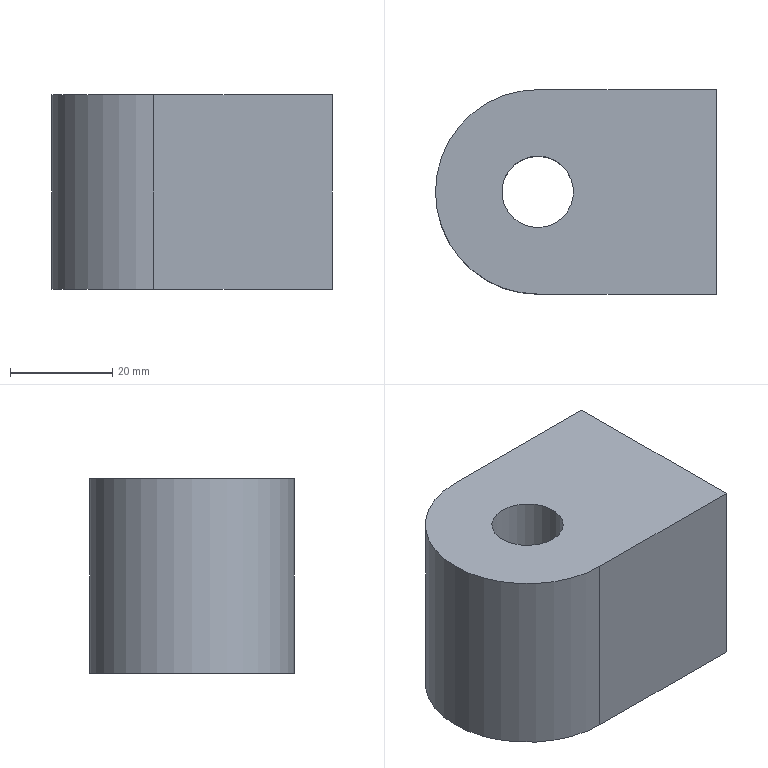Component | NX | Z_AXIS_LEADSCREW_NUT | 1 solid | 15 faces | box 55 x 40 x 38 mm | volume 69853 mm3 | cylinder 6 | plane 5 | cone 4 | commonest cylinder face diameters 5 x4 40 x1 14 x1
STEP:
#1=CARTESIAN_POINT('',(0.,0.,0.));
#2=DIRECTION('',(0.,0.,1.));
#3=DIRECTION('',(1.,0.,0.));
#4=AXIS2_PLACEMENT_3D('',#1,#2,#3);
#5=CARTESIAN_POINT('',(660.689,-130.302,-1073.));
#6=VERTEX_POINT('',#5);
#7=CARTESIAN_POINT('',(625.689,-130.302,-1073.));
#8=VERTEX_POINT('',#7);
#9=CARTESIAN_POINT('',(660.689,-130.302,-1073.));
#10=DIRECTION('',(-1.,0.,0.));
#11=VECTOR('',#10,1.);
#12=LINE('',#9,#11);
#13=CARTESIAN_POINT('',(660.689,-130.302,-1035.));
#14=DIRECTION('',(0.,-1.,0.));
#15=DIRECTION('',(0.,0.,-1.));
#16=AXIS2_PLACEMENT_3D('',#13,#14,#15);
#17=PLANE('',#16);
#18=CARTESIAN_POINT('',(38.,0.));
#19=DIRECTION('',(0.,-1.));
#20=VECTOR('',#19,1.);
#21=LINE('',#18,#20);
#22=(GEOMETRIC_REPRESENTATION_CONTEXT(2)PARAMETRIC_REPRESENTATION_CONTEXT()REPRESENTATION_CONTEXT('',''));
#23=DEFINITIONAL_REPRESENTATION('',(#21),#22);
#24=PCURVE('',#17,#23);
#25=CARTESIAN_POINT('',(625.689,-150.302,-1073.));
#26=DIRECTION('',(0.,0.,1.));
#27=DIRECTION('',(0.,-1.,0.));
#28=AXIS2_PLACEMENT_3D('',#25,#26,#27);
#29=PLANE('',#28);
#30=CARTESIAN_POINT('',(-20.,35.));
#31=DIRECTION('',(0.,-1.));
#32=VECTOR('',#31,1.);
#33=LINE('',#30,#32);
#34=(GEOMETRIC_REPRESENTATION_CONTEXT(2)PARAMETRIC_REPRESENTATION_CONTEXT()REPRESENTATION_CONTEXT('',''));
#35=DEFINITIONAL_REPRESENTATION('',(#33),#34);
#36=PCURVE('',#29,#35);
#37=SURFACE_CURVE('',#12,(#24,#36),.PCURVE_S1.);
#38=EDGE_CURVE('',#6,#8,#37,.T.);
#39=ORIENTED_EDGE('',*,*,#38,.T.);
#40=CARTESIAN_POINT('',(625.689,-130.302,-1035.));
#41=VERTEX_POINT('',#40);
#42=CARTESIAN_POINT('',(625.689,-130.302,-1035.));
#43=DIRECTION('',(0.,0.,-1.));
#44=VECTOR('',#43,1.);
#45=LINE('',#42,#44);
#46=CARTESIAN_POINT('',(0.,-35.));
#47=DIRECTION('',(1.,0.));
#48=VECTOR('',#47,1.);
#49=LINE('',#46,#48);
#50=(GEOMETRIC_REPRESENTATION_CONTEXT(2)PARAMETRIC_REPRESENTATION_CONTEXT()REPRESENTATION_CONTEXT('',''));
#51=DEFINITIONAL_REPRESENTATION('',(#49),#50);
#52=PCURVE('',#17,#51);
#53=CARTESIAN_POINT('',(625.689,-150.302,-1035.));
#54=DIRECTION('',(0.,0.,-1.));
#55=DIRECTION('',(0.,1.,0.));
#56=AXIS2_PLACEMENT_3D('',#53,#54,#55);
#57=CYLINDRICAL_SURFACE('',#56,20.);
#58=CARTESIAN_POINT('',(6.283,0.));
#59=DIRECTION('',(0.,1.));
#60=VECTOR('',#59,1.);
#61=LINE('',#58,#60);
#62=(GEOMETRIC_REPRESENTATION_CONTEXT(2)PARAMETRIC_REPRESENTATION_CONTEXT()REPRESENTATION_CONTEXT('',''));
#63=DEFINITIONAL_REPRESENTATION('',(#61),#62);
#64=PCURVE('',#57,#63);
#65=SURFACE_CURVE('',#45,(#52,#64),.PCURVE_S1.);
#66=EDGE_CURVE('',#41,#8,#65,.T.);
#67=ORIENTED_EDGE('',*,*,#66,.F.);
#68=CARTESIAN_POINT('',(660.689,-130.302,-1035.));
#69=VERTEX_POINT('',#68);
#70=CARTESIAN_POINT('',(660.689,-130.302,-1035.));
#71=DIRECTION('',(-1.,0.,0.));
#72=VECTOR('',#71,1.);
#73=LINE('',#70,#72);
#74=CARTESIAN_POINT('',(0.,0.));
#75=DIRECTION('',(0.,-1.));
#76=VECTOR('',#75,1.);
#77=LINE('',#74,#76);
#78=(GEOMETRIC_REPRESENTATION_CONTEXT(2)PARAMETRIC_REPRESENTATION_CONTEXT()REPRESENTATION_CONTEXT('',''));
#79=DEFINITIONAL_REPRESENTATION('',(#77),#78);
#80=PCURVE('',#17,#79);
#81=CARTESIAN_POINT('',(625.689,-150.302,-1035.));
#82=DIRECTION('',(0.,0.,1.));
#83=DIRECTION('',(0.,-1.,0.));
#84=AXIS2_PLACEMENT_3D('',#81,#82,#83);
#85=PLANE('',#84);
#86=CARTESIAN_POINT('',(-20.,35.));
#87=DIRECTION('',(0.,-1.));
#88=VECTOR('',#87,1.);
#89=LINE('',#86,#88);
#90=(GEOMETRIC_REPRESENTATION_CONTEXT(2)PARAMETRIC_REPRESENTATION_CONTEXT()REPRESENTATION_CONTEXT('',''));
#91=DEFINITIONAL_REPRESENTATION('',(#89),#90);
#92=PCURVE('',#85,#91);
#93=SURFACE_CURVE('',#73,(#80,#92),.PCURVE_S1.);
#94=EDGE_CURVE('',#69,#41,#93,.T.);
#95=ORIENTED_EDGE('',*,*,#94,.F.);
#96=CARTESIAN_POINT('',(660.689,-130.302,-1035.));
#97=DIRECTION('',(0.,0.,-1.));
#98=VECTOR('',#97,1.);
#99=LINE('',#96,#98);
#100=CARTESIAN_POINT('',(0.,0.));
#101=DIRECTION('',(1.,0.));
#102=VECTOR('',#101,1.);
#103=LINE('',#100,#102);
#104=(GEOMETRIC_REPRESENTATION_CONTEXT(2)PARAMETRIC_REPRESENTATION_CONTEXT()REPRESENTATION_CONTEXT('',''));
#105=DEFINITIONAL_REPRESENTATION('',(#103),#104);
#106=PCURVE('',#17,#105);
#107=CARTESIAN_POINT('',(660.689,-170.302,-1035.));
#108=DIRECTION('',(-1.,0.,0.));
#109=DIRECTION('',(0.,0.,-1.));
#110=AXIS2_PLACEMENT_3D('',#107,#108,#109);
#111=PLANE('',#110);
#112=CARTESIAN_POINT('',(0.,-40.));
#113=DIRECTION('',(1.,0.));
#114=VECTOR('',#113,1.);
#115=LINE('',#112,#114);
#116=(GEOMETRIC_REPRESENTATION_CONTEXT(2)PARAMETRIC_REPRESENTATION_CONTEXT()REPRESENTATION_CONTEXT('',''));
#117=DEFINITIONAL_REPRESENTATION('',(#115),#116);
#118=PCURVE('',#111,#117);
#119=SURFACE_CURVE('',#99,(#106,#118),.PCURVE_S1.);
#120=EDGE_CURVE('',#69,#6,#119,.T.);
#121=ORIENTED_EDGE('',*,*,#120,.T.);
#122=EDGE_LOOP('',(#39,#67,#95,#121));
#123=FACE_BOUND('',#122,.T.);
#124=ADVANCED_FACE('',(#123),#17,.F.);
#125=CARTESIAN_POINT('',(625.689,-170.302,-1073.));
#126=VERTEX_POINT('',#125);
#127=CARTESIAN_POINT('',(625.689,-150.302,-1073.));
#128=DIRECTION('',(0.,0.,1.));
#129=DIRECTION('',(0.,-1.,0.));
#130=AXIS2_PLACEMENT_3D('',#127,#128,#129);
#131=CIRCLE('',#130,20.);
#132=CARTESIAN_POINT('',(9.425,38.));
#133=DIRECTION('',(-1.,0.));
#134=VECTOR('',#133,1.);
#135=LINE('',#132,#134);
#136=(GEOMETRIC_REPRESENTATION_CONTEXT(2)PARAMETRIC_REPRESENTATION_CONTEXT()REPRESENTATION_CONTEXT('',''));
#137=DEFINITIONAL_REPRESENTATION('',(#135),#136);
#138=PCURVE('',#57,#137);
#139=CARTESIAN_POINT('',(0.,0.));
#140=DIRECTION('',(1.,0.));
#141=AXIS2_PLACEMENT_2D('',#139,#140);
#142=CIRCLE('',#141,20.);
#143=(GEOMETRIC_REPRESENTATION_CONTEXT(2)PARAMETRIC_REPRESENTATION_CONTEXT()REPRESENTATION_CONTEXT('',''));
#144=DEFINITIONAL_REPRESENTATION('',(#142),#143);
#145=PCURVE('',#29,#144);
#146=SURFACE_CURVE('',#131,(#138,#145),.PCURVE_S1.);
#147=EDGE_CURVE('',#8,#126,#146,.T.);
#148=ORIENTED_EDGE('',*,*,#147,.T.);
#149=CARTESIAN_POINT('',(625.689,-170.302,-1035.));
#150=VERTEX_POINT('',#149);
#151=CARTESIAN_POINT('',(625.689,-170.302,-1035.));
#152=DIRECTION('',(0.,0.,-1.));
#153=VECTOR('',#152,1.);
#154=LINE('',#151,#153);
#155=CARTESIAN_POINT('',(3.142,0.));
#156=DIRECTION('',(0.,1.));
#157=VECTOR('',#156,1.);
#158=LINE('',#155,#157);
#159=(GEOMETRIC_REPRESENTATION_CONTEXT(2)PARAMETRIC_REPRESENTATION_CONTEXT()REPRESENTATION_CONTEXT('',''));
#160=DEFINITIONAL_REPRESENTATION('',(#158),#159);
#161=PCURVE('',#57,#160);
#162=CARTESIAN_POINT('',(625.689,-170.302,-1035.));
#163=DIRECTION('',(0.,1.,0.));
#164=DIRECTION('',(0.,0.,1.));
#165=AXIS2_PLACEMENT_3D('',#162,#163,#164);
#166=PLANE('',#165);
#167=CARTESIAN_POINT('',(0.,0.));
#168=DIRECTION('',(-1.,0.));
#169=VECTOR('',#168,1.);
#170=LINE('',#167,#169);
#171=(GEOMETRIC_REPRESENTATION_CONTEXT(2)PARAMETRIC_REPRESENTATION_CONTEXT()REPRESENTATION_CONTEXT('',''));
#172=DEFINITIONAL_REPRESENTATION('',(#170),#171);
#173=PCURVE('',#166,#172);
#174=SURFACE_CURVE('',#154,(#161,#173),.PCURVE_S1.);
#175=EDGE_CURVE('',#150,#126,#174,.T.);
#176=ORIENTED_EDGE('',*,*,#175,.F.);
#177=CARTESIAN_POINT('',(625.689,-150.302,-1035.));
#178=DIRECTION('',(0.,0.,1.));
#179=DIRECTION('',(0.,-1.,0.));
#180=AXIS2_PLACEMENT_3D('',#177,#178,#179);
#181=CIRCLE('',#180,20.);
#182=CARTESIAN_POINT('',(9.425,0.));
#183=DIRECTION('',(-1.,0.));
#184=VECTOR('',#183,1.);
#185=LINE('',#182,#184);
#186=(GEOMETRIC_REPRESENTATION_CONTEXT(2)PARAMETRIC_REPRESENTATION_CONTEXT()REPRESENTATION_CONTEXT('',''));
#187=DEFINITIONAL_REPRESENTATION('',(#185),#186);
#188=PCURVE('',#57,#187);
#189=CARTESIAN_POINT('',(0.,0.));
#190=DIRECTION('',(1.,0.));
#191=AXIS2_PLACEMENT_2D('',#189,#190);
#192=CIRCLE('',#191,20.);
#193=(GEOMETRIC_REPRESENTATION_CONTEXT(2)PARAMETRIC_REPRESENTATION_CONTEXT()REPRESENTATION_CONTEXT('',''));
#194=DEFINITIONAL_REPRESENTATION('',(#192),#193);
#195=PCURVE('',#85,#194);
#196=SURFACE_CURVE('',#181,(#188,#195),.PCURVE_S1.);
#197=EDGE_CURVE('',#41,#150,#196,.T.);
#198=ORIENTED_EDGE('',*,*,#197,.F.);
#199=ORIENTED_EDGE('',*,*,#66,.T.);
#200=EDGE_LOOP('',(#148,#176,#198,#199));
#201=FACE_BOUND('',#200,.T.);
#202=ADVANCED_FACE('',(#201),#57,.T.);
#203=CARTESIAN_POINT('',(660.689,-170.302,-1073.));
#204=VERTEX_POINT('',#203);
#205=CARTESIAN_POINT('',(625.689,-170.302,-1073.));
#206=DIRECTION('',(1.,0.,0.));
#207=VECTOR('',#206,1.);
#208=LINE('',#205,#207);
#209=CARTESIAN_POINT('',(-38.,0.));
#210=DIRECTION('',(0.,1.));
#211=VECTOR('',#210,1.);
#212=LINE('',#209,#211);
#213=(GEOMETRIC_REPRESENTATION_CONTEXT(2)PARAMETRIC_REPRESENTATION_CONTEXT()REPRESENTATION_CONTEXT('',''));
#214=DEFINITIONAL_REPRESENTATION('',(#212),#213);
#215=PCURVE('',#166,#214);
#216=CARTESIAN_POINT('',(20.,0.));
#217=DIRECTION('',(0.,1.));
#218=VECTOR('',#217,1.);
#219=LINE('',#216,#218);
#220=(GEOMETRIC_REPRESENTATION_CONTEXT(2)PARAMETRIC_REPRESENTATION_CONTEXT()REPRESENTATION_CONTEXT('',''));
#221=DEFINITIONAL_REPRESENTATION('',(#219),#220);
#222=PCURVE('',#29,#221);
#223=SURFACE_CURVE('',#208,(#215,#222),.PCURVE_S1.);
#224=EDGE_CURVE('',#126,#204,#223,.T.);
#225=ORIENTED_EDGE('',*,*,#224,.T.);
#226=CARTESIAN_POINT('',(660.689,-170.302,-1035.));
#227=VERTEX_POINT('',#226);
#228=CARTESIAN_POINT('',(660.689,-170.302,-1035.));
#229=DIRECTION('',(0.,0.,-1.));
#230=VECTOR('',#229,1.);
#231=LINE('',#228,#230);
#232=CARTESIAN_POINT('',(0.,35.));
#233=DIRECTION('',(-1.,0.));
#234=VECTOR('',#233,1.);
#235=LINE('',#232,#234);
#236=(GEOMETRIC_REPRESENTATION_CONTEXT(2)PARAMETRIC_REPRESENTATION_CONTEXT()REPRESENTATION_CONTEXT('',''));
#237=DEFINITIONAL_REPRESENTATION('',(#235),#236);
#238=PCURVE('',#166,#237);
#239=CARTESIAN_POINT('',(0.,0.));
#240=DIRECTION('',(1.,0.));
#241=VECTOR('',#240,1.);
#242=LINE('',#239,#241);
#243=(GEOMETRIC_REPRESENTATION_CONTEXT(2)PARAMETRIC_REPRESENTATION_CONTEXT()REPRESENTATION_CONTEXT('',''));
#244=DEFINITIONAL_REPRESENTATION('',(#242),#243);
#245=PCURVE('',#111,#244);
#246=SURFACE_CURVE('',#231,(#238,#245),.PCURVE_S1.);
#247=EDGE_CURVE('',#227,#204,#246,.T.);
#248=ORIENTED_EDGE('',*,*,#247,.F.);
#249=CARTESIAN_POINT('',(625.689,-170.302,-1035.));
#250=DIRECTION('',(1.,0.,0.));
#251=VECTOR('',#250,1.);
#252=LINE('',#249,#251);
#253=CARTESIAN_POINT('',(0.,0.));
#254=DIRECTION('',(0.,1.));
#255=VECTOR('',#254,1.);
#256=LINE('',#253,#255);
#257=(GEOMETRIC_REPRESENTATION_CONTEXT(2)PARAMETRIC_REPRESENTATION_CONTEXT()REPRESENTATION_CONTEXT('',''));
#258=DEFINITIONAL_REPRESENTATION('',(#256),#257);
#259=PCURVE('',#166,#258);
#260=CARTESIAN_POINT('',(20.,0.));
#261=DIRECTION('',(0.,1.));
#262=VECTOR('',#261,1.);
#263=LINE('',#260,#262);
#264=(GEOMETRIC_REPRESENTATION_CONTEXT(2)PARAMETRIC_REPRESENTATION_CONTEXT()REPRESENTATION_CONTEXT('',''));
#265=DEFINITIONAL_REPRESENTATION('',(#263),#264);
#266=PCURVE('',#85,#265);
#267=SURFACE_CURVE('',#252,(#259,#266),.PCURVE_S1.);
#268=EDGE_CURVE('',#150,#227,#267,.T.);
#269=ORIENTED_EDGE('',*,*,#268,.F.);
#270=ORIENTED_EDGE('',*,*,#175,.T.);
#271=EDGE_LOOP('',(#225,#248,#269,#270));
#272=FACE_BOUND('',#271,.T.);
#273=ADVANCED_FACE('',(#272),#166,.F.);
#274=CARTESIAN_POINT('',(660.689,-163.302,-1043.5));
#275=VERTEX_POINT('',#274);
#276=CARTESIAN_POINT('',(660.689,-163.302,-1041.));
#277=DIRECTION('',(-1.,0.,0.));
#278=DIRECTION('',(0.,0.,-1.));
#279=AXIS2_PLACEMENT_3D('',#276,#277,#278);
#280=CIRCLE('',#279,2.5);
#281=CARTESIAN_POINT('',(6.,-7.));
#282=DIRECTION('',(1.,0.));
#283=AXIS2_PLACEMENT_2D('',#281,#282);
#284=CIRCLE('',#283,2.5);
#285=(GEOMETRIC_REPRESENTATION_CONTEXT(2)PARAMETRIC_REPRESENTATION_CONTEXT()REPRESENTATION_CONTEXT('',''));
#286=DEFINITIONAL_REPRESENTATION('',(#284),#285);
#287=PCURVE('',#111,#286);
#288=CARTESIAN_POINT('',(660.689,-163.302,-1041.));
#289=DIRECTION('',(-1.,0.,0.));
#290=DIRECTION('',(0.,0.,-1.));
#291=AXIS2_PLACEMENT_3D('',#288,#289,#290);
#292=CYLINDRICAL_SURFACE('',#291,2.5);
#293=CARTESIAN_POINT('',(0.,0.));
#294=DIRECTION('',(1.,0.));
#295=VECTOR('',#294,1.);
#296=LINE('',#293,#295);
#297=(GEOMETRIC_REPRESENTATION_CONTEXT(2)PARAMETRIC_REPRESENTATION_CONTEXT()REPRESENTATION_CONTEXT('',''));
#298=DEFINITIONAL_REPRESENTATION('',(#296),#297);
#299=PCURVE('',#292,#298);
#300=SURFACE_CURVE('',#280,(#287,#299),.PCURVE_S1.);
#301=EDGE_CURVE('',#275,#275,#300,.T.);
#302=ORIENTED_EDGE('',*,*,#301,.T.);
#303=EDGE_LOOP('',(#302));
#304=FACE_BOUND('',#303,.T.);
#305=CARTESIAN_POINT('',(660.689,-163.302,-1069.5));
#306=VERTEX_POINT('',#305);
#307=CARTESIAN_POINT('',(660.689,-163.302,-1067.));
#308=DIRECTION('',(-1.,0.,0.));
#309=DIRECTION('',(0.,0.,-1.));
#310=AXIS2_PLACEMENT_3D('',#307,#308,#309);
#311=CIRCLE('',#310,2.5);
#312=CARTESIAN_POINT('',(32.,-7.));
#313=DIRECTION('',(1.,0.));
#314=AXIS2_PLACEMENT_2D('',#312,#313);
#315=CIRCLE('',#314,2.5);
#316=(GEOMETRIC_REPRESENTATION_CONTEXT(2)PARAMETRIC_REPRESENTATION_CONTEXT()REPRESENTATION_CONTEXT('',''));
#317=DEFINITIONAL_REPRESENTATION('',(#315),#316);
#318=PCURVE('',#111,#317);
#319=CARTESIAN_POINT('',(660.689,-163.302,-1067.));
#320=DIRECTION('',(-1.,0.,0.));
#321=DIRECTION('',(0.,0.,-1.));
#322=AXIS2_PLACEMENT_3D('',#319,#320,#321);
#323=CYLINDRICAL_SURFACE('',#322,2.5);
#324=CARTESIAN_POINT('',(0.,0.));
#325=DIRECTION('',(1.,0.));
#326=VECTOR('',#325,1.);
#327=LINE('',#324,#326);
#328=(GEOMETRIC_REPRESENTATION_CONTEXT(2)PARAMETRIC_REPRESENTATION_CONTEXT()REPRESENTATION_CONTEXT('',''));
#329=DEFINITIONAL_REPRESENTATION('',(#327),#328);
#330=PCURVE('',#323,#329);
#331=SURFACE_CURVE('',#311,(#318,#330),.PCURVE_S1.);
#332=EDGE_CURVE('',#306,#306,#331,.T.);
#333=ORIENTED_EDGE('',*,*,#332,.T.);
#334=EDGE_LOOP('',(#333));
#335=FACE_BOUND('',#334,.T.);
#336=CARTESIAN_POINT('',(660.689,-137.302,-1043.5));
#337=VERTEX_POINT('',#336);
#338=CARTESIAN_POINT('',(660.689,-137.302,-1041.));
#339=DIRECTION('',(-1.,0.,0.));
#340=DIRECTION('',(0.,0.,-1.));
#341=AXIS2_PLACEMENT_3D('',#338,#339,#340);
#342=CIRCLE('',#341,2.5);
#343=CARTESIAN_POINT('',(6.,-33.));
#344=DIRECTION('',(1.,0.));
#345=AXIS2_PLACEMENT_2D('',#343,#344);
#346=CIRCLE('',#345,2.5);
#347=(GEOMETRIC_REPRESENTATION_CONTEXT(2)PARAMETRIC_REPRESENTATION_CONTEXT()REPRESENTATION_CONTEXT('',''));
#348=DEFINITIONAL_REPRESENTATION('',(#346),#347);
#349=PCURVE('',#111,#348);
#350=CARTESIAN_POINT('',(660.689,-137.302,-1041.));
#351=DIRECTION('',(-1.,0.,0.));
#352=DIRECTION('',(0.,0.,-1.));
#353=AXIS2_PLACEMENT_3D('',#350,#351,#352);
#354=CYLINDRICAL_SURFACE('',#353,2.5);
#355=CARTESIAN_POINT('',(0.,0.));
#356=DIRECTION('',(1.,0.));
#357=VECTOR('',#356,1.);
#358=LINE('',#355,#357);
#359=(GEOMETRIC_REPRESENTATION_CONTEXT(2)PARAMETRIC_REPRESENTATION_CONTEXT()REPRESENTATION_CONTEXT('',''));
#360=DEFINITIONAL_REPRESENTATION('',(#358),#359);
#361=PCURVE('',#354,#360);
#362=SURFACE_CURVE('',#342,(#349,#361),.PCURVE_S1.);
#363=EDGE_CURVE('',#337,#337,#362,.T.);
#364=ORIENTED_EDGE('',*,*,#363,.T.);
#365=EDGE_LOOP('',(#364));
#366=FACE_BOUND('',#365,.T.);
#367=CARTESIAN_POINT('',(660.689,-137.302,-1069.5));
#368=VERTEX_POINT('',#367);
#369=CARTESIAN_POINT('',(660.689,-137.302,-1067.));
#370=DIRECTION('',(-1.,0.,0.));
#371=DIRECTION('',(0.,0.,-1.));
#372=AXIS2_PLACEMENT_3D('',#369,#370,#371);
#373=CIRCLE('',#372,2.5);
#374=CARTESIAN_POINT('',(32.,-33.));
#375=DIRECTION('',(1.,0.));
#376=AXIS2_PLACEMENT_2D('',#374,#375);
#377=CIRCLE('',#376,2.5);
#378=(GEOMETRIC_REPRESENTATION_CONTEXT(2)PARAMETRIC_REPRESENTATION_CONTEXT()REPRESENTATION_CONTEXT('',''));
#379=DEFINITIONAL_REPRESENTATION('',(#377),#378);
#380=PCURVE('',#111,#379);
#381=CARTESIAN_POINT('',(660.689,-137.302,-1067.));
#382=DIRECTION('',(-1.,0.,0.));
#383=DIRECTION('',(0.,0.,-1.));
#384=AXIS2_PLACEMENT_3D('',#381,#382,#383);
#385=CYLINDRICAL_SURFACE('',#384,2.5);
#386=CARTESIAN_POINT('',(0.,0.));
#387=DIRECTION('',(1.,0.));
#388=VECTOR('',#387,1.);
#389=LINE('',#386,#388);
#390=(GEOMETRIC_REPRESENTATION_CONTEXT(2)PARAMETRIC_REPRESENTATION_CONTEXT()REPRESENTATION_CONTEXT('',''));
#391=DEFINITIONAL_REPRESENTATION('',(#389),#390);
#392=PCURVE('',#385,#391);
#393=SURFACE_CURVE('',#373,(#380,#392),.PCURVE_S1.);
#394=EDGE_CURVE('',#368,#368,#393,.T.);
#395=ORIENTED_EDGE('',*,*,#394,.T.);
#396=EDGE_LOOP('',(#395));
#397=FACE_BOUND('',#396,.T.);
#398=CARTESIAN_POINT('',(660.689,-170.302,-1073.));
#399=DIRECTION('',(0.,1.,0.));
#400=VECTOR('',#399,1.);
#401=LINE('',#398,#400);
#402=CARTESIAN_POINT('',(38.,0.));
#403=DIRECTION('',(0.,-1.));
#404=VECTOR('',#403,1.);
#405=LINE('',#402,#404);
#406=(GEOMETRIC_REPRESENTATION_CONTEXT(2)PARAMETRIC_REPRESENTATION_CONTEXT()REPRESENTATION_CONTEXT('',''));
#407=DEFINITIONAL_REPRESENTATION('',(#405),#406);
#408=PCURVE('',#111,#407);
#409=CARTESIAN_POINT('',(20.,35.));
#410=DIRECTION('',(-1.,0.));
#411=VECTOR('',#410,1.);
#412=LINE('',#409,#411);
#413=(GEOMETRIC_REPRESENTATION_CONTEXT(2)PARAMETRIC_REPRESENTATION_CONTEXT()REPRESENTATION_CONTEXT('',''));
#414=DEFINITIONAL_REPRESENTATION('',(#412),#413);
#415=PCURVE('',#29,#414);
#416=SURFACE_CURVE('',#401,(#408,#415),.PCURVE_S1.);
#417=EDGE_CURVE('',#204,#6,#416,.T.);
#418=ORIENTED_EDGE('',*,*,#417,.T.);
#419=ORIENTED_EDGE('',*,*,#120,.F.);
#420=CARTESIAN_POINT('',(660.689,-170.302,-1035.));
#421=DIRECTION('',(0.,1.,0.));
#422=VECTOR('',#421,1.);
#423=LINE('',#420,#422);
#424=CARTESIAN_POINT('',(0.,0.));
#425=DIRECTION('',(0.,-1.));
#426=VECTOR('',#425,1.);
#427=LINE('',#424,#426);
#428=(GEOMETRIC_REPRESENTATION_CONTEXT(2)PARAMETRIC_REPRESENTATION_CONTEXT()REPRESENTATION_CONTEXT('',''));
#429=DEFINITIONAL_REPRESENTATION('',(#427),#428);
#430=PCURVE('',#111,#429);
#431=CARTESIAN_POINT('',(20.,35.));
#432=DIRECTION('',(-1.,0.));
#433=VECTOR('',#432,1.);
#434=LINE('',#431,#433);
#435=(GEOMETRIC_REPRESENTATION_CONTEXT(2)PARAMETRIC_REPRESENTATION_CONTEXT()REPRESENTATION_CONTEXT('',''));
#436=DEFINITIONAL_REPRESENTATION('',(#434),#435);
#437=PCURVE('',#85,#436);
#438=SURFACE_CURVE('',#423,(#430,#437),.PCURVE_S1.);
#439=EDGE_CURVE('',#227,#69,#438,.T.);
#440=ORIENTED_EDGE('',*,*,#439,.F.);
#441=ORIENTED_EDGE('',*,*,#247,.T.);
#442=EDGE_LOOP('',(#418,#419,#440,#441));
#443=FACE_BOUND('',#442,.T.);
#444=ADVANCED_FACE('',(#304,#335,#366,#397,#443),#111,.F.);
#445=CARTESIAN_POINT('',(625.689,-157.302,-1035.));
#446=VERTEX_POINT('',#445);
#447=CARTESIAN_POINT('',(625.689,-150.302,-1035.));
#448=DIRECTION('',(0.,0.,1.));
#449=DIRECTION('',(0.,-1.,0.));
#450=AXIS2_PLACEMENT_3D('',#447,#448,#449);
#451=CIRCLE('',#450,7.);
#452=CARTESIAN_POINT('',(625.689,-150.302,-1035.));
#453=DIRECTION('',(0.,0.,-1.));
#454=DIRECTION('',(0.,1.,0.));
#455=AXIS2_PLACEMENT_3D('',#452,#453,#454);
#456=CYLINDRICAL_SURFACE('',#455,7.);
#457=CARTESIAN_POINT('',(9.425,0.));
#458=DIRECTION('',(-1.,0.));
#459=VECTOR('',#458,1.);
#460=LINE('',#457,#459);
#461=(GEOMETRIC_REPRESENTATION_CONTEXT(2)PARAMETRIC_REPRESENTATION_CONTEXT()REPRESENTATION_CONTEXT('',''));
#462=DEFINITIONAL_REPRESENTATION('',(#460),#461);
#463=PCURVE('',#456,#462);
#464=CARTESIAN_POINT('',(0.,0.));
#465=DIRECTION('',(1.,0.));
#466=AXIS2_PLACEMENT_2D('',#464,#465);
#467=CIRCLE('',#466,7.);
#468=(GEOMETRIC_REPRESENTATION_CONTEXT(2)PARAMETRIC_REPRESENTATION_CONTEXT()REPRESENTATION_CONTEXT('',''));
#469=DEFINITIONAL_REPRESENTATION('',(#467),#468);
#470=PCURVE('',#85,#469);
#471=SURFACE_CURVE('',#451,(#463,#470),.PCURVE_S1.);
#472=EDGE_CURVE('',#446,#446,#471,.T.);
#473=ORIENTED_EDGE('',*,*,#472,.F.);
#474=CARTESIAN_POINT('',(625.689,-157.302,-1073.));
#475=VERTEX_POINT('',#474);
#476=CARTESIAN_POINT('',(625.689,-157.302,-1035.));
#477=CARTESIAN_POINT('',(625.689,-157.302,-1073.));
#478=B_SPLINE_CURVE_WITH_KNOTS('',1,(#476,#477),.UNSPECIFIED.,.F.,.F.,(2,2),(0.,38.),.PIECEWISE_BEZIER_KNOTS.);
#479=CARTESIAN_POINT('',(9.425,0.));
#480=DIRECTION('',(0.,1.));
#481=VECTOR('',#480,1.);
#482=LINE('',#479,#481);
#483=(GEOMETRIC_REPRESENTATION_CONTEXT(2)PARAMETRIC_REPRESENTATION_CONTEXT()REPRESENTATION_CONTEXT('',''));
#484=DEFINITIONAL_REPRESENTATION('',(#482),#483);
#485=PCURVE('',#456,#484);
#486=CARTESIAN_POINT('',(3.142,0.));
#487=DIRECTION('',(0.,1.));
#488=VECTOR('',#487,1.);
#489=LINE('',#486,#488);
#490=(GEOMETRIC_REPRESENTATION_CONTEXT(2)PARAMETRIC_REPRESENTATION_CONTEXT()REPRESENTATION_CONTEXT('',''));
#491=DEFINITIONAL_REPRESENTATION('',(#489),#490);
#492=PCURVE('',#456,#491);
#493=SEAM_CURVE('',#478,(#485,#492),.PCURVE_S1.);
#494=EDGE_CURVE('',#446,#475,#493,.T.);
#495=ORIENTED_EDGE('',*,*,#494,.T.);
#496=CARTESIAN_POINT('',(625.689,-150.302,-1073.));
#497=DIRECTION('',(0.,0.,1.));
#498=DIRECTION('',(0.,-1.,0.));
#499=AXIS2_PLACEMENT_3D('',#496,#497,#498);
#500=CIRCLE('',#499,7.);
#501=CARTESIAN_POINT('',(9.425,38.));
#502=DIRECTION('',(-1.,0.));
#503=VECTOR('',#502,1.);
#504=LINE('',#501,#503);
#505=(GEOMETRIC_REPRESENTATION_CONTEXT(2)PARAMETRIC_REPRESENTATION_CONTEXT()REPRESENTATION_CONTEXT('',''));
#506=DEFINITIONAL_REPRESENTATION('',(#504),#505);
#507=PCURVE('',#456,#506);
#508=CARTESIAN_POINT('',(0.,0.));
#509=DIRECTION('',(1.,0.));
#510=AXIS2_PLACEMENT_2D('',#508,#509);
#511=CIRCLE('',#510,7.);
#512=(GEOMETRIC_REPRESENTATION_CONTEXT(2)PARAMETRIC_REPRESENTATION_CONTEXT()REPRESENTATION_CONTEXT('',''));
#513=DEFINITIONAL_REPRESENTATION('',(#511),#512);
#514=PCURVE('',#29,#513);
#515=SURFACE_CURVE('',#500,(#507,#514),.PCURVE_S1.);
#516=EDGE_CURVE('',#475,#475,#515,.T.);
#517=ORIENTED_EDGE('',*,*,#516,.T.);
#518=ORIENTED_EDGE('',*,*,#494,.F.);
#519=EDGE_LOOP('',(#473,#495,#517,#518));
#520=FACE_BOUND('',#519,.F.);
#521=ADVANCED_FACE('',(#520),#456,.F.);
#522=ORIENTED_EDGE('',*,*,#94,.T.);
#523=ORIENTED_EDGE('',*,*,#197,.T.);
#524=ORIENTED_EDGE('',*,*,#268,.T.);
#525=ORIENTED_EDGE('',*,*,#439,.T.);
#526=EDGE_LOOP('',(#522,#523,#524,#525));
#527=FACE_BOUND('',#526,.T.);
#528=ORIENTED_EDGE('',*,*,#472,.F.);
#529=EDGE_LOOP('',(#528));
#530=FACE_BOUND('',#529,.T.);
#531=ADVANCED_FACE('',(#527,#530),#85,.T.);
#532=ORIENTED_EDGE('',*,*,#38,.F.);
#533=ORIENTED_EDGE('',*,*,#417,.F.);
#534=ORIENTED_EDGE('',*,*,#224,.F.);
#535=ORIENTED_EDGE('',*,*,#147,.F.);
#536=EDGE_LOOP('',(#532,#533,#534,#535));
#537=FACE_BOUND('',#536,.T.);
#538=ORIENTED_EDGE('',*,*,#516,.T.);
#539=EDGE_LOOP('',(#538));
#540=FACE_BOUND('',#539,.T.);
#541=ADVANCED_FACE('',(#537,#540),#29,.F.);
#542=CARTESIAN_POINT('',(643.689,-137.302,-1064.5));
#543=VERTEX_POINT('',#542);
#544=CARTESIAN_POINT('',(643.689,-137.302,-1069.5));
#545=VERTEX_POINT('',#544);
#546=CARTESIAN_POINT('',(643.689,-137.302,-1067.));
#547=DIRECTION('',(1.,0.,0.));
#548=DIRECTION('',(0.,0.,-1.));
#549=AXIS2_PLACEMENT_3D('',#546,#547,#548);
#550=CIRCLE('',#549,2.5);
#551=CARTESIAN_POINT('',(643.689,-137.302,-1067.));
#552=DIRECTION('',(1.,0.,0.));
#553=DIRECTION('',(0.,0.,1.));
#554=AXIS2_PLACEMENT_3D('',#551,#552,#553);
#555=CONICAL_SURFACE('',#554,2.5,1.047);
#556=CARTESIAN_POINT('',(-3.142,0.));
#557=DIRECTION('',(1.,0.));
#558=VECTOR('',#557,1.);
#559=LINE('',#556,#558);
#560=(GEOMETRIC_REPRESENTATION_CONTEXT(2)PARAMETRIC_REPRESENTATION_CONTEXT()REPRESENTATION_CONTEXT('',''));
#561=DEFINITIONAL_REPRESENTATION('',(#559),#560);
#562=PCURVE('',#555,#561);
#563=CARTESIAN_POINT('',(6.283,17.));
#564=DIRECTION('',(-1.,0.));
#565=VECTOR('',#564,1.);
#566=LINE('',#563,#565);
#567=(GEOMETRIC_REPRESENTATION_CONTEXT(2)PARAMETRIC_REPRESENTATION_CONTEXT()REPRESENTATION_CONTEXT('',''));
#568=DEFINITIONAL_REPRESENTATION('',(#566),#567);
#569=PCURVE('',#385,#568);
#570=SURFACE_CURVE('',#550,(#562,#569),.PCURVE_S1.);
#571=EDGE_CURVE('',#543,#545,#570,.T.);
#572=ORIENTED_EDGE('',*,*,#571,.F.);
#573=CARTESIAN_POINT('',(642.246,-137.302,-1067.));
#574=VERTEX_POINT('',#573);
#575=CARTESIAN_POINT('',(642.246,-137.302,-1067.));
#576=CARTESIAN_POINT('',(643.689,-137.302,-1064.5));
#577=B_SPLINE_CURVE_WITH_KNOTS('',1,(#575,#576),.UNSPECIFIED.,.F.,.F.,(2,2),(-2.887,0.),.PIECEWISE_BEZIER_KNOTS.);
#578=CARTESIAN_POINT('',(0.,0.));
#579=DIRECTION('',(0.,1.));
#580=VECTOR('',#579,1.);
#581=LINE('',#578,#580);
#582=(GEOMETRIC_REPRESENTATION_CONTEXT(2)PARAMETRIC_REPRESENTATION_CONTEXT()REPRESENTATION_CONTEXT('',''));
#583=DEFINITIONAL_REPRESENTATION('',(#581),#582);
#584=PCURVE('',#555,#583);
#585=CARTESIAN_POINT('',(6.283,0.));
#586=DIRECTION('',(0.,1.));
#587=VECTOR('',#586,1.);
#588=LINE('',#585,#587);
#589=(GEOMETRIC_REPRESENTATION_CONTEXT(2)PARAMETRIC_REPRESENTATION_CONTEXT()REPRESENTATION_CONTEXT('',''));
#590=DEFINITIONAL_REPRESENTATION('',(#588),#589);
#591=PCURVE('',#555,#590);
#592=SEAM_CURVE('',#577,(#584,#591),.PCURVE_S1.);
#593=EDGE_CURVE('',#574,#543,#592,.T.);
#594=ORIENTED_EDGE('',*,*,#593,.F.);
#595=ORIENTED_EDGE('',*,*,#593,.T.);
#596=CARTESIAN_POINT('',(643.689,-137.302,-1067.));
#597=DIRECTION('',(1.,0.,0.));
#598=DIRECTION('',(0.,0.,-1.));
#599=AXIS2_PLACEMENT_3D('',#596,#597,#598);
#600=CIRCLE('',#599,2.5);
#601=CARTESIAN_POINT('',(3.142,0.));
#602=DIRECTION('',(1.,0.));
#603=VECTOR('',#602,1.);
#604=LINE('',#601,#603);
#605=(GEOMETRIC_REPRESENTATION_CONTEXT(2)PARAMETRIC_REPRESENTATION_CONTEXT()REPRESENTATION_CONTEXT('',''));
#606=DEFINITIONAL_REPRESENTATION('',(#604),#605);
#607=PCURVE('',#555,#606);
#608=CARTESIAN_POINT('',(6.283,17.));
#609=DIRECTION('',(-1.,0.));
#610=VECTOR('',#609,1.);
#611=LINE('',#608,#610);
#612=(GEOMETRIC_REPRESENTATION_CONTEXT(2)PARAMETRIC_REPRESENTATION_CONTEXT()REPRESENTATION_CONTEXT('',''));
#613=DEFINITIONAL_REPRESENTATION('',(#611),#612);
#614=PCURVE('',#385,#613);
#615=SURFACE_CURVE('',#600,(#607,#614),.PCURVE_S1.);
#616=EDGE_CURVE('',#545,#543,#615,.T.);
#617=ORIENTED_EDGE('',*,*,#616,.F.);
#618=EDGE_LOOP('',(#572,#594,#595,#617));
#619=FACE_BOUND('',#618,.F.);
#620=ADVANCED_FACE('',(#619),#555,.F.);
#621=ORIENTED_EDGE('',*,*,#571,.T.);
#622=CARTESIAN_POINT('',(660.689,-137.302,-1069.5));
#623=CARTESIAN_POINT('',(643.689,-137.302,-1069.5));
#624=B_SPLINE_CURVE_WITH_KNOTS('',1,(#622,#623),.UNSPECIFIED.,.F.,.F.,(2,2),(0.,17.),.PIECEWISE_BEZIER_KNOTS.);
#625=CARTESIAN_POINT('',(0.,0.));
#626=DIRECTION('',(0.,1.));
#627=VECTOR('',#626,1.);
#628=LINE('',#625,#627);
#629=(GEOMETRIC_REPRESENTATION_CONTEXT(2)PARAMETRIC_REPRESENTATION_CONTEXT()REPRESENTATION_CONTEXT('',''));
#630=DEFINITIONAL_REPRESENTATION('',(#628),#629);
#631=PCURVE('',#385,#630);
#632=CARTESIAN_POINT('',(6.283,0.));
#633=DIRECTION('',(0.,1.));
#634=VECTOR('',#633,1.);
#635=LINE('',#632,#634);
#636=(GEOMETRIC_REPRESENTATION_CONTEXT(2)PARAMETRIC_REPRESENTATION_CONTEXT()REPRESENTATION_CONTEXT('',''));
#637=DEFINITIONAL_REPRESENTATION('',(#635),#636);
#638=PCURVE('',#385,#637);
#639=SEAM_CURVE('',#624,(#631,#638),.PCURVE_S1.);
#640=EDGE_CURVE('',#368,#545,#639,.T.);
#641=ORIENTED_EDGE('',*,*,#640,.F.);
#642=ORIENTED_EDGE('',*,*,#394,.T.);
#643=ORIENTED_EDGE('',*,*,#640,.T.);
#644=ORIENTED_EDGE('',*,*,#616,.T.);
#645=EDGE_LOOP('',(#621,#641,#642,#643,#644));
#646=FACE_BOUND('',#645,.F.);
#647=ADVANCED_FACE('',(#646),#385,.F.);
#648=CARTESIAN_POINT('',(643.689,-137.302,-1038.5));
#649=VERTEX_POINT('',#648);
#650=CARTESIAN_POINT('',(643.689,-137.302,-1043.5));
#651=VERTEX_POINT('',#650);
#652=CARTESIAN_POINT('',(643.689,-137.302,-1041.));
#653=DIRECTION('',(1.,0.,0.));
#654=DIRECTION('',(0.,0.,-1.));
#655=AXIS2_PLACEMENT_3D('',#652,#653,#654);
#656=CIRCLE('',#655,2.5);
#657=CARTESIAN_POINT('',(643.689,-137.302,-1041.));
#658=DIRECTION('',(1.,0.,0.));
#659=DIRECTION('',(0.,0.,1.));
#660=AXIS2_PLACEMENT_3D('',#657,#658,#659);
#661=CONICAL_SURFACE('',#660,2.5,1.047);
#662=CARTESIAN_POINT('',(-3.142,0.));
#663=DIRECTION('',(1.,0.));
#664=VECTOR('',#663,1.);
#665=LINE('',#662,#664);
#666=(GEOMETRIC_REPRESENTATION_CONTEXT(2)PARAMETRIC_REPRESENTATION_CONTEXT()REPRESENTATION_CONTEXT('',''));
#667=DEFINITIONAL_REPRESENTATION('',(#665),#666);
#668=PCURVE('',#661,#667);
#669=CARTESIAN_POINT('',(6.283,17.));
#670=DIRECTION('',(-1.,0.));
#671=VECTOR('',#670,1.);
#672=LINE('',#669,#671);
#673=(GEOMETRIC_REPRESENTATION_CONTEXT(2)PARAMETRIC_REPRESENTATION_CONTEXT()REPRESENTATION_CONTEXT('',''));
#674=DEFINITIONAL_REPRESENTATION('',(#672),#673);
#675=PCURVE('',#354,#674);
#676=SURFACE_CURVE('',#656,(#668,#675),.PCURVE_S1.);
#677=EDGE_CURVE('',#649,#651,#676,.T.);
#678=ORIENTED_EDGE('',*,*,#677,.F.);
#679=CARTESIAN_POINT('',(642.246,-137.302,-1041.));
#680=VERTEX_POINT('',#679);
#681=CARTESIAN_POINT('',(642.246,-137.302,-1041.));
#682=CARTESIAN_POINT('',(643.689,-137.302,-1038.5));
#683=B_SPLINE_CURVE_WITH_KNOTS('',1,(#681,#682),.UNSPECIFIED.,.F.,.F.,(2,2),(-2.887,0.),.PIECEWISE_BEZIER_KNOTS.);
#684=CARTESIAN_POINT('',(0.,0.));
#685=DIRECTION('',(0.,1.));
#686=VECTOR('',#685,1.);
#687=LINE('',#684,#686);
#688=(GEOMETRIC_REPRESENTATION_CONTEXT(2)PARAMETRIC_REPRESENTATION_CONTEXT()REPRESENTATION_CONTEXT('',''));
#689=DEFINITIONAL_REPRESENTATION('',(#687),#688);
#690=PCURVE('',#661,#689);
#691=CARTESIAN_POINT('',(6.283,0.));
#692=DIRECTION('',(0.,1.));
#693=VECTOR('',#692,1.);
#694=LINE('',#691,#693);
#695=(GEOMETRIC_REPRESENTATION_CONTEXT(2)PARAMETRIC_REPRESENTATION_CONTEXT()REPRESENTATION_CONTEXT('',''));
#696=DEFINITIONAL_REPRESENTATION('',(#694),#695);
#697=PCURVE('',#661,#696);
#698=SEAM_CURVE('',#683,(#690,#697),.PCURVE_S1.);
#699=EDGE_CURVE('',#680,#649,#698,.T.);
#700=ORIENTED_EDGE('',*,*,#699,.F.);
#701=ORIENTED_EDGE('',*,*,#699,.T.);
#702=CARTESIAN_POINT('',(643.689,-137.302,-1041.));
#703=DIRECTION('',(1.,0.,0.));
#704=DIRECTION('',(0.,0.,-1.));
#705=AXIS2_PLACEMENT_3D('',#702,#703,#704);
#706=CIRCLE('',#705,2.5);
#707=CARTESIAN_POINT('',(3.142,0.));
#708=DIRECTION('',(1.,0.));
#709=VECTOR('',#708,1.);
#710=LINE('',#707,#709);
#711=(GEOMETRIC_REPRESENTATION_CONTEXT(2)PARAMETRIC_REPRESENTATION_CONTEXT()REPRESENTATION_CONTEXT('',''));
#712=DEFINITIONAL_REPRESENTATION('',(#710),#711);
#713=PCURVE('',#661,#712);
#714=CARTESIAN_POINT('',(6.283,17.));
#715=DIRECTION('',(-1.,0.));
#716=VECTOR('',#715,1.);
#717=LINE('',#714,#716);
#718=(GEOMETRIC_REPRESENTATION_CONTEXT(2)PARAMETRIC_REPRESENTATION_CONTEXT()REPRESENTATION_CONTEXT('',''));
#719=DEFINITIONAL_REPRESENTATION('',(#717),#718);
#720=PCURVE('',#354,#719);
#721=SURFACE_CURVE('',#706,(#713,#720),.PCURVE_S1.);
#722=EDGE_CURVE('',#651,#649,#721,.T.);
#723=ORIENTED_EDGE('',*,*,#722,.F.);
#724=EDGE_LOOP('',(#678,#700,#701,#723));
#725=FACE_BOUND('',#724,.F.);
#726=ADVANCED_FACE('',(#725),#661,.F.);
#727=ORIENTED_EDGE('',*,*,#677,.T.);
#728=CARTESIAN_POINT('',(660.689,-137.302,-1043.5));
#729=CARTESIAN_POINT('',(643.689,-137.302,-1043.5));
#730=B_SPLINE_CURVE_WITH_KNOTS('',1,(#728,#729),.UNSPECIFIED.,.F.,.F.,(2,2),(0.,17.),.PIECEWISE_BEZIER_KNOTS.);
#731=CARTESIAN_POINT('',(0.,0.));
#732=DIRECTION('',(0.,1.));
#733=VECTOR('',#732,1.);
#734=LINE('',#731,#733);
#735=(GEOMETRIC_REPRESENTATION_CONTEXT(2)PARAMETRIC_REPRESENTATION_CONTEXT()REPRESENTATION_CONTEXT('',''));
#736=DEFINITIONAL_REPRESENTATION('',(#734),#735);
#737=PCURVE('',#354,#736);
#738=CARTESIAN_POINT('',(6.283,0.));
#739=DIRECTION('',(0.,1.));
#740=VECTOR('',#739,1.);
#741=LINE('',#738,#740);
#742=(GEOMETRIC_REPRESENTATION_CONTEXT(2)PARAMETRIC_REPRESENTATION_CONTEXT()REPRESENTATION_CONTEXT('',''));
#743=DEFINITIONAL_REPRESENTATION('',(#741),#742);
#744=PCURVE('',#354,#743);
#745=SEAM_CURVE('',#730,(#737,#744),.PCURVE_S1.);
#746=EDGE_CURVE('',#337,#651,#745,.T.);
#747=ORIENTED_EDGE('',*,*,#746,.F.);
#748=ORIENTED_EDGE('',*,*,#363,.T.);
#749=ORIENTED_EDGE('',*,*,#746,.T.);
#750=ORIENTED_EDGE('',*,*,#722,.T.);
#751=EDGE_LOOP('',(#727,#747,#748,#749,#750));
#752=FACE_BOUND('',#751,.F.);
#753=ADVANCED_FACE('',(#752),#354,.F.);
#754=CARTESIAN_POINT('',(643.689,-163.302,-1064.5));
#755=VERTEX_POINT('',#754);
#756=CARTESIAN_POINT('',(643.689,-163.302,-1069.5));
#757=VERTEX_POINT('',#756);
#758=CARTESIAN_POINT('',(643.689,-163.302,-1067.));
#759=DIRECTION('',(1.,0.,0.));
#760=DIRECTION('',(0.,0.,-1.));
#761=AXIS2_PLACEMENT_3D('',#758,#759,#760);
#762=CIRCLE('',#761,2.5);
#763=CARTESIAN_POINT('',(643.689,-163.302,-1067.));
#764=DIRECTION('',(1.,0.,0.));
#765=DIRECTION('',(0.,0.,1.));
#766=AXIS2_PLACEMENT_3D('',#763,#764,#765);
#767=CONICAL_SURFACE('',#766,2.5,1.047);
#768=CARTESIAN_POINT('',(-3.142,0.));
#769=DIRECTION('',(1.,0.));
#770=VECTOR('',#769,1.);
#771=LINE('',#768,#770);
#772=(GEOMETRIC_REPRESENTATION_CONTEXT(2)PARAMETRIC_REPRESENTATION_CONTEXT()REPRESENTATION_CONTEXT('',''));
#773=DEFINITIONAL_REPRESENTATION('',(#771),#772);
#774=PCURVE('',#767,#773);
#775=CARTESIAN_POINT('',(6.283,17.));
#776=DIRECTION('',(-1.,0.));
#777=VECTOR('',#776,1.);
#778=LINE('',#775,#777);
#779=(GEOMETRIC_REPRESENTATION_CONTEXT(2)PARAMETRIC_REPRESENTATION_CONTEXT()REPRESENTATION_CONTEXT('',''));
#780=DEFINITIONAL_REPRESENTATION('',(#778),#779);
#781=PCURVE('',#323,#780);
#782=SURFACE_CURVE('',#762,(#774,#781),.PCURVE_S1.);
#783=EDGE_CURVE('',#755,#757,#782,.T.);
#784=ORIENTED_EDGE('',*,*,#783,.F.);
#785=CARTESIAN_POINT('',(642.246,-163.302,-1067.));
#786=VERTEX_POINT('',#785);
#787=CARTESIAN_POINT('',(642.246,-163.302,-1067.));
#788=CARTESIAN_POINT('',(643.689,-163.302,-1064.5));
#789=B_SPLINE_CURVE_WITH_KNOTS('',1,(#787,#788),.UNSPECIFIED.,.F.,.F.,(2,2),(-2.887,0.),.PIECEWISE_BEZIER_KNOTS.);
#790=CARTESIAN_POINT('',(0.,0.));
#791=DIRECTION('',(0.,1.));
#792=VECTOR('',#791,1.);
#793=LINE('',#790,#792);
#794=(GEOMETRIC_REPRESENTATION_CONTEXT(2)PARAMETRIC_REPRESENTATION_CONTEXT()REPRESENTATION_CONTEXT('',''));
#795=DEFINITIONAL_REPRESENTATION('',(#793),#794);
#796=PCURVE('',#767,#795);
#797=CARTESIAN_POINT('',(6.283,0.));
#798=DIRECTION('',(0.,1.));
#799=VECTOR('',#798,1.);
#800=LINE('',#797,#799);
#801=(GEOMETRIC_REPRESENTATION_CONTEXT(2)PARAMETRIC_REPRESENTATION_CONTEXT()REPRESENTATION_CONTEXT('',''));
#802=DEFINITIONAL_REPRESENTATION('',(#800),#801);
#803=PCURVE('',#767,#802);
#804=SEAM_CURVE('',#789,(#796,#803),.PCURVE_S1.);
#805=EDGE_CURVE('',#786,#755,#804,.T.);
#806=ORIENTED_EDGE('',*,*,#805,.F.);
#807=ORIENTED_EDGE('',*,*,#805,.T.);
#808=CARTESIAN_POINT('',(643.689,-163.302,-1067.));
#809=DIRECTION('',(1.,0.,0.));
#810=DIRECTION('',(0.,0.,-1.));
#811=AXIS2_PLACEMENT_3D('',#808,#809,#810);
#812=CIRCLE('',#811,2.5);
#813=CARTESIAN_POINT('',(3.142,0.));
#814=DIRECTION('',(1.,0.));
#815=VECTOR('',#814,1.);
#816=LINE('',#813,#815);
#817=(GEOMETRIC_REPRESENTATION_CONTEXT(2)PARAMETRIC_REPRESENTATION_CONTEXT()REPRESENTATION_CONTEXT('',''));
#818=DEFINITIONAL_REPRESENTATION('',(#816),#817);
#819=PCURVE('',#767,#818);
#820=CARTESIAN_POINT('',(6.283,17.));
#821=DIRECTION('',(-1.,0.));
#822=VECTOR('',#821,1.);
#823=LINE('',#820,#822);
#824=(GEOMETRIC_REPRESENTATION_CONTEXT(2)PARAMETRIC_REPRESENTATION_CONTEXT()REPRESENTATION_CONTEXT('',''));
#825=DEFINITIONAL_REPRESENTATION('',(#823),#824);
#826=PCURVE('',#323,#825);
#827=SURFACE_CURVE('',#812,(#819,#826),.PCURVE_S1.);
#828=EDGE_CURVE('',#757,#755,#827,.T.);
#829=ORIENTED_EDGE('',*,*,#828,.F.);
#830=EDGE_LOOP('',(#784,#806,#807,#829));
#831=FACE_BOUND('',#830,.F.);
#832=ADVANCED_FACE('',(#831),#767,.F.);
#833=ORIENTED_EDGE('',*,*,#783,.T.);
#834=CARTESIAN_POINT('',(660.689,-163.302,-1069.5));
#835=CARTESIAN_POINT('',(643.689,-163.302,-1069.5));
#836=B_SPLINE_CURVE_WITH_KNOTS('',1,(#834,#835),.UNSPECIFIED.,.F.,.F.,(2,2),(0.,17.),.PIECEWISE_BEZIER_KNOTS.);
#837=CARTESIAN_POINT('',(0.,0.));
#838=DIRECTION('',(0.,1.));
#839=VECTOR('',#838,1.);
#840=LINE('',#837,#839);
#841=(GEOMETRIC_REPRESENTATION_CONTEXT(2)PARAMETRIC_REPRESENTATION_CONTEXT()REPRESENTATION_CONTEXT('',''));
#842=DEFINITIONAL_REPRESENTATION('',(#840),#841);
#843=PCURVE('',#323,#842);
#844=CARTESIAN_POINT('',(6.283,0.));
#845=DIRECTION('',(0.,1.));
#846=VECTOR('',#845,1.);
#847=LINE('',#844,#846);
#848=(GEOMETRIC_REPRESENTATION_CONTEXT(2)PARAMETRIC_REPRESENTATION_CONTEXT()REPRESENTATION_CONTEXT('',''));
#849=DEFINITIONAL_REPRESENTATION('',(#847),#848);
#850=PCURVE('',#323,#849);
#851=SEAM_CURVE('',#836,(#843,#850),.PCURVE_S1.);
#852=EDGE_CURVE('',#306,#757,#851,.T.);
#853=ORIENTED_EDGE('',*,*,#852,.F.);
#854=ORIENTED_EDGE('',*,*,#332,.T.);
#855=ORIENTED_EDGE('',*,*,#852,.T.);
#856=ORIENTED_EDGE('',*,*,#828,.T.);
#857=EDGE_LOOP('',(#833,#853,#854,#855,#856));
#858=FACE_BOUND('',#857,.F.);
#859=ADVANCED_FACE('',(#858),#323,.F.);
#860=CARTESIAN_POINT('',(643.689,-163.302,-1038.5));
#861=VERTEX_POINT('',#860);
#862=CARTESIAN_POINT('',(643.689,-163.302,-1043.5));
#863=VERTEX_POINT('',#862);
#864=CARTESIAN_POINT('',(643.689,-163.302,-1041.));
#865=DIRECTION('',(1.,0.,0.));
#866=DIRECTION('',(0.,0.,-1.));
#867=AXIS2_PLACEMENT_3D('',#864,#865,#866);
#868=CIRCLE('',#867,2.5);
#869=CARTESIAN_POINT('',(643.689,-163.302,-1041.));
#870=DIRECTION('',(1.,0.,0.));
#871=DIRECTION('',(0.,0.,1.));
#872=AXIS2_PLACEMENT_3D('',#869,#870,#871);
#873=CONICAL_SURFACE('',#872,2.5,1.047);
#874=CARTESIAN_POINT('',(-3.142,0.));
#875=DIRECTION('',(1.,0.));
#876=VECTOR('',#875,1.);
#877=LINE('',#874,#876);
#878=(GEOMETRIC_REPRESENTATION_CONTEXT(2)PARAMETRIC_REPRESENTATION_CONTEXT()REPRESENTATION_CONTEXT('',''));
#879=DEFINITIONAL_REPRESENTATION('',(#877),#878);
#880=PCURVE('',#873,#879);
#881=CARTESIAN_POINT('',(6.283,17.));
#882=DIRECTION('',(-1.,0.));
#883=VECTOR('',#882,1.);
#884=LINE('',#881,#883);
#885=(GEOMETRIC_REPRESENTATION_CONTEXT(2)PARAMETRIC_REPRESENTATION_CONTEXT()REPRESENTATION_CONTEXT('',''));
#886=DEFINITIONAL_REPRESENTATION('',(#884),#885);
#887=PCURVE('',#292,#886);
#888=SURFACE_CURVE('',#868,(#880,#887),.PCURVE_S1.);
#889=EDGE_CURVE('',#861,#863,#888,.T.);
#890=ORIENTED_EDGE('',*,*,#889,.F.);
#891=CARTESIAN_POINT('',(642.246,-163.302,-1041.));
#892=VERTEX_POINT('',#891);
#893=CARTESIAN_POINT('',(642.246,-163.302,-1041.));
#894=CARTESIAN_POINT('',(643.689,-163.302,-1038.5));
#895=B_SPLINE_CURVE_WITH_KNOTS('',1,(#893,#894),.UNSPECIFIED.,.F.,.F.,(2,2),(-2.887,0.),.PIECEWISE_BEZIER_KNOTS.);
#896=CARTESIAN_POINT('',(0.,0.));
#897=DIRECTION('',(0.,1.));
#898=VECTOR('',#897,1.);
#899=LINE('',#896,#898);
#900=(GEOMETRIC_REPRESENTATION_CONTEXT(2)PARAMETRIC_REPRESENTATION_CONTEXT()REPRESENTATION_CONTEXT('',''));
#901=DEFINITIONAL_REPRESENTATION('',(#899),#900);
#902=PCURVE('',#873,#901);
#903=CARTESIAN_POINT('',(6.283,0.));
#904=DIRECTION('',(0.,1.));
#905=VECTOR('',#904,1.);
#906=LINE('',#903,#905);
#907=(GEOMETRIC_REPRESENTATION_CONTEXT(2)PARAMETRIC_REPRESENTATION_CONTEXT()REPRESENTATION_CONTEXT('',''));
#908=DEFINITIONAL_REPRESENTATION('',(#906),#907);
#909=PCURVE('',#873,#908);
#910=SEAM_CURVE('',#895,(#902,#909),.PCURVE_S1.);
#911=EDGE_CURVE('',#892,#861,#910,.T.);
#912=ORIENTED_EDGE('',*,*,#911,.F.);
#913=ORIENTED_EDGE('',*,*,#911,.T.);
#914=CARTESIAN_POINT('',(643.689,-163.302,-1041.));
#915=DIRECTION('',(1.,0.,0.));
#916=DIRECTION('',(0.,0.,-1.));
#917=AXIS2_PLACEMENT_3D('',#914,#915,#916);
#918=CIRCLE('',#917,2.5);
#919=CARTESIAN_POINT('',(3.142,0.));
#920=DIRECTION('',(1.,0.));
#921=VECTOR('',#920,1.);
#922=LINE('',#919,#921);
#923=(GEOMETRIC_REPRESENTATION_CONTEXT(2)PARAMETRIC_REPRESENTATION_CONTEXT()REPRESENTATION_CONTEXT('',''));
#924=DEFINITIONAL_REPRESENTATION('',(#922),#923);
#925=PCURVE('',#873,#924);
#926=CARTESIAN_POINT('',(6.283,17.));
#927=DIRECTION('',(-1.,0.));
#928=VECTOR('',#927,1.);
#929=LINE('',#926,#928);
#930=(GEOMETRIC_REPRESENTATION_CONTEXT(2)PARAMETRIC_REPRESENTATION_CONTEXT()REPRESENTATION_CONTEXT('',''));
#931=DEFINITIONAL_REPRESENTATION('',(#929),#930);
#932=PCURVE('',#292,#931);
#933=SURFACE_CURVE('',#918,(#925,#932),.PCURVE_S1.);
#934=EDGE_CURVE('',#863,#861,#933,.T.);
#935=ORIENTED_EDGE('',*,*,#934,.F.);
#936=EDGE_LOOP('',(#890,#912,#913,#935));
#937=FACE_BOUND('',#936,.F.);
#938=ADVANCED_FACE('',(#937),#873,.F.);
#939=ORIENTED_EDGE('',*,*,#889,.T.);
#940=CARTESIAN_POINT('',(660.689,-163.302,-1043.5));
#941=CARTESIAN_POINT('',(643.689,-163.302,-1043.5));
#942=B_SPLINE_CURVE_WITH_KNOTS('',1,(#940,#941),.UNSPECIFIED.,.F.,.F.,(2,2),(0.,17.),.PIECEWISE_BEZIER_KNOTS.);
#943=CARTESIAN_POINT('',(0.,0.));
#944=DIRECTION('',(0.,1.));
#945=VECTOR('',#944,1.);
#946=LINE('',#943,#945);
#947=(GEOMETRIC_REPRESENTATION_CONTEXT(2)PARAMETRIC_REPRESENTATION_CONTEXT()REPRESENTATION_CONTEXT('',''));
#948=DEFINITIONAL_REPRESENTATION('',(#946),#947);
#949=PCURVE('',#292,#948);
#950=CARTESIAN_POINT('',(6.283,0.));
#951=DIRECTION('',(0.,1.));
#952=VECTOR('',#951,1.);
#953=LINE('',#950,#952);
#954=(GEOMETRIC_REPRESENTATION_CONTEXT(2)PARAMETRIC_REPRESENTATION_CONTEXT()REPRESENTATION_CONTEXT('',''));
#955=DEFINITIONAL_REPRESENTATION('',(#953),#954);
#956=PCURVE('',#292,#955);
#957=SEAM_CURVE('',#942,(#949,#956),.PCURVE_S1.);
#958=EDGE_CURVE('',#275,#863,#957,.T.);
#959=ORIENTED_EDGE('',*,*,#958,.F.);
#960=ORIENTED_EDGE('',*,*,#301,.T.);
#961=ORIENTED_EDGE('',*,*,#958,.T.);
#962=ORIENTED_EDGE('',*,*,#934,.T.);
#963=EDGE_LOOP('',(#939,#959,#960,#961,#962));
#964=FACE_BOUND('',#963,.F.);
#965=ADVANCED_FACE('',(#964),#292,.F.);
#966=CLOSED_SHELL('',(#124,#202,#273,#444,#521,#531,#541,#620,#647,#726,#753,#832,#859,#938,#965));
#967=MANIFOLD_SOLID_BREP('',#966);
#968=(LENGTH_UNIT()NAMED_UNIT(*)SI_UNIT(.MILLI.,.METRE.));
#969=UNCERTAINTY_MEASURE_WITH_UNIT(LENGTH_MEASURE(0.000005),#968,'','');
#970=(NAMED_UNIT(*)PLANE_ANGLE_UNIT()SI_UNIT($,.RADIAN.));
#971=(NAMED_UNIT(*)SI_UNIT($,.STERADIAN.)SOLID_ANGLE_UNIT());
#972=(GEOMETRIC_REPRESENTATION_CONTEXT(3)GLOBAL_UNCERTAINTY_ASSIGNED_CONTEXT((#969))GLOBAL_UNIT_ASSIGNED_CONTEXT((#968,#970,#971))REPRESENTATION_CONTEXT('',''));
#973=ADVANCED_BREP_SHAPE_REPRESENTATION('',(#4,#967),#972);